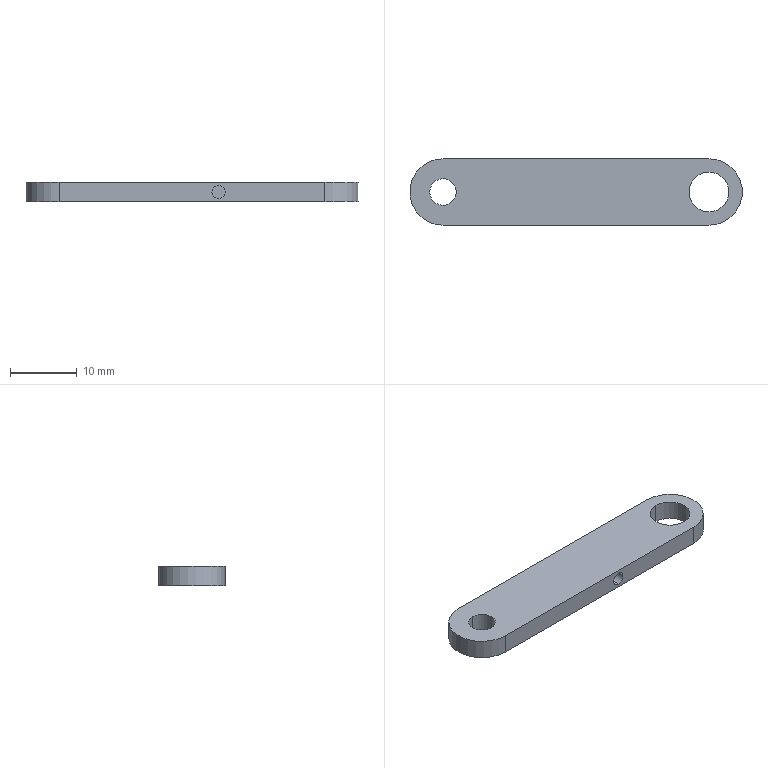CAM job | Mastercam | mm | 8 operations | part box 50 x 10 x 3
1. Facing | 12 - 12 平铣刀
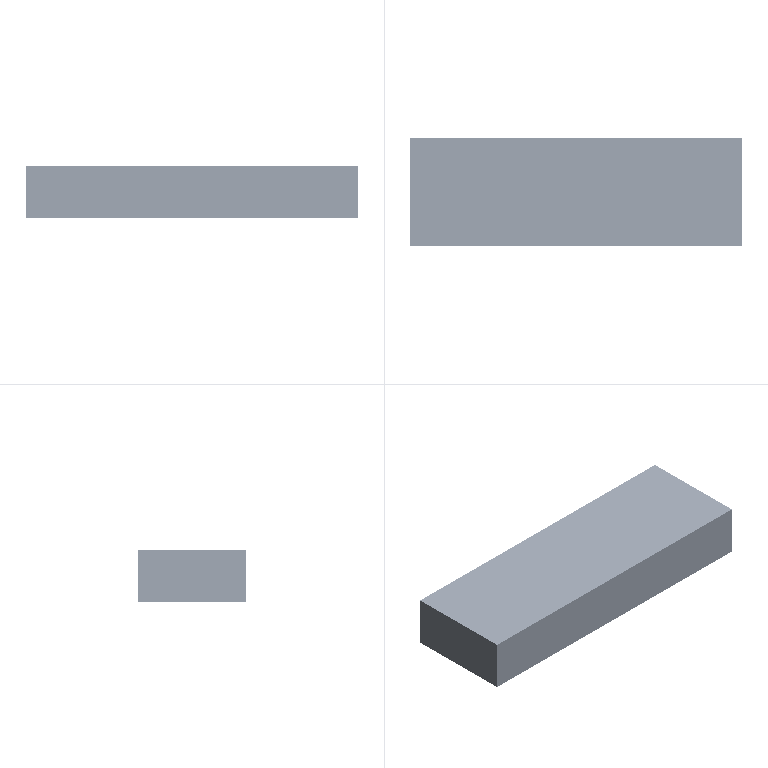2. Contour (Ramp) | 12 - 12 平铣刀
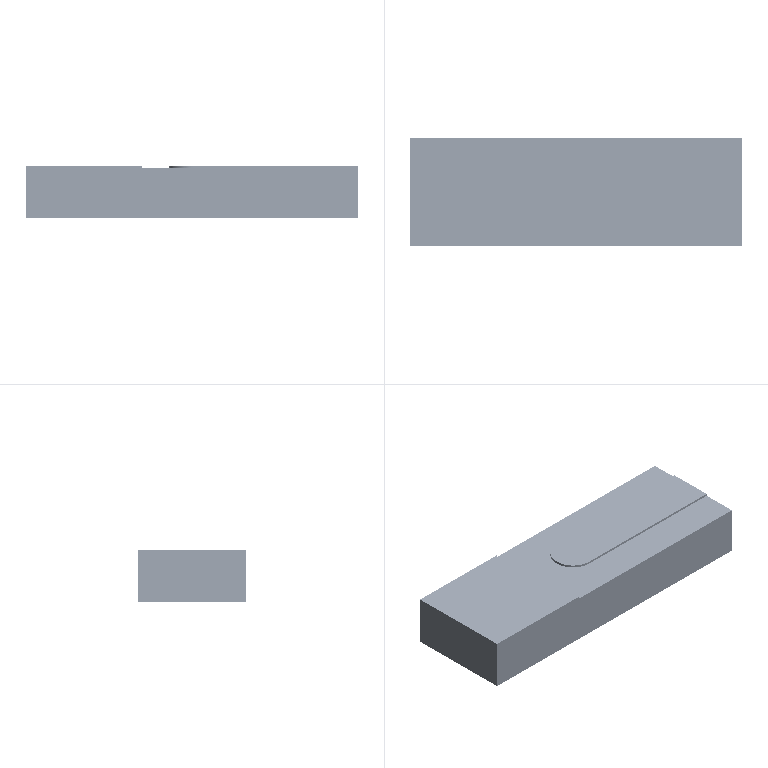3. Contour (2D) | 12 - 12 平铣刀
4. Drill/Counterbore | 7 - 4 倒角刀
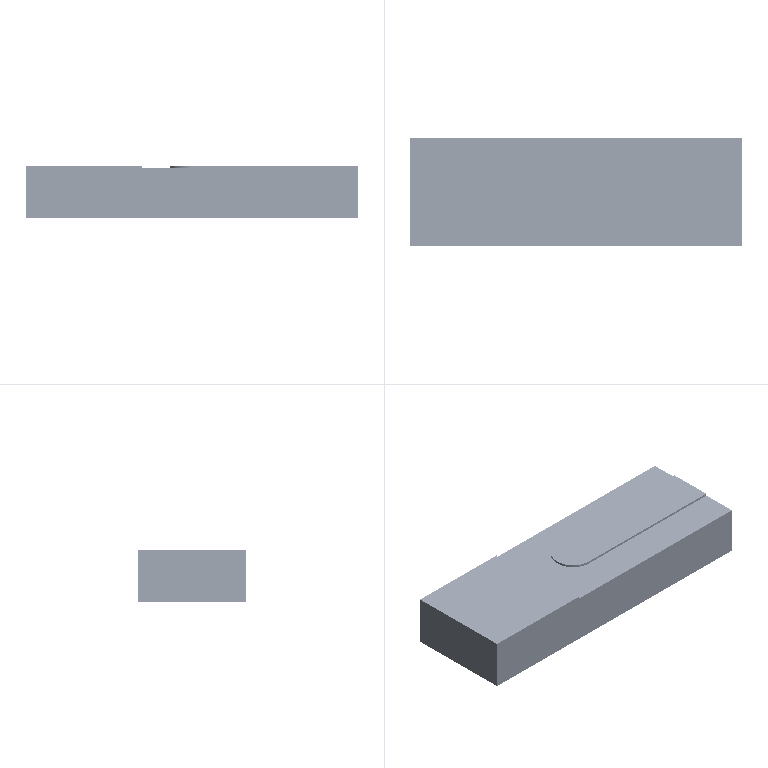5. Contour (2D chamfer) | 7 - 4 倒角刀
6. Facing | 12 - 12 平铣刀
7. Contour (2D chamfer) | 7 - 4 倒角刀
8. Drill/Counterbore | 7 - 4 倒角刀